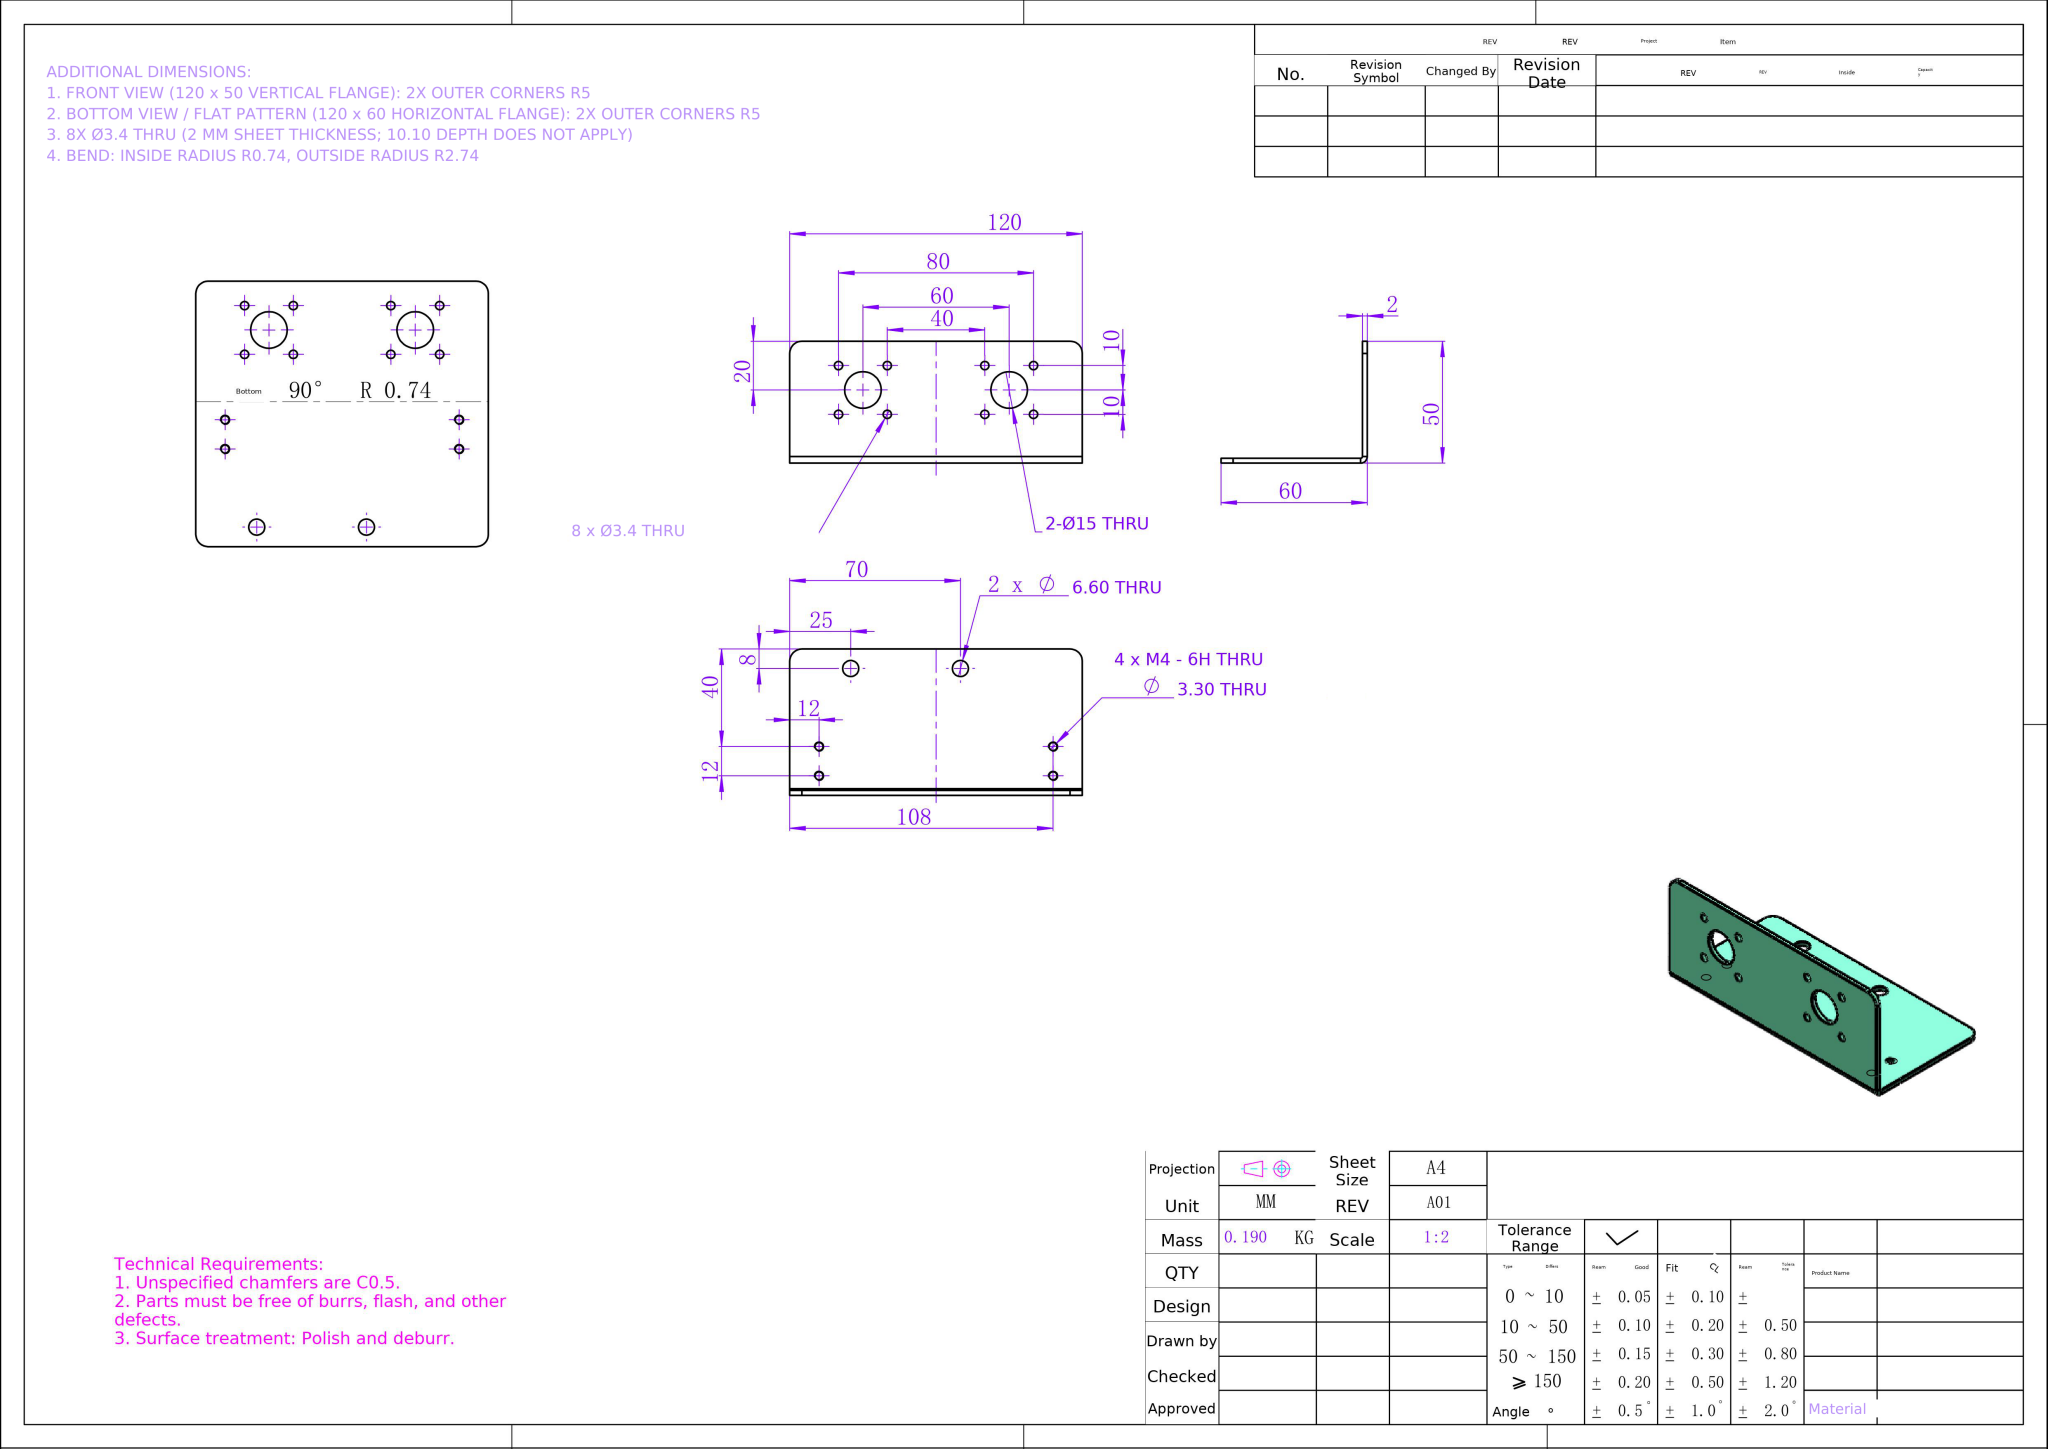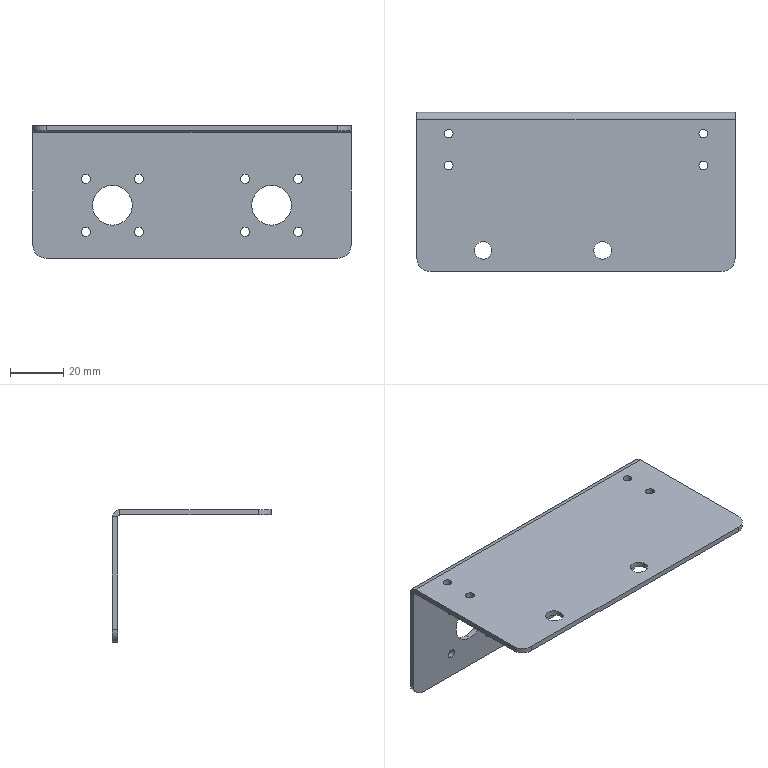Part | NX | mm | 1 solid | 50 faces | box 120 x 60 x 50 mm | volume 24641 mm3 | cylinder 38 | plane 12 | commonest cylinder face diameters 3.4 x16 3.3 x8 15 x4 6.6 x4 10 x4 5.473 x1 1.473 x1